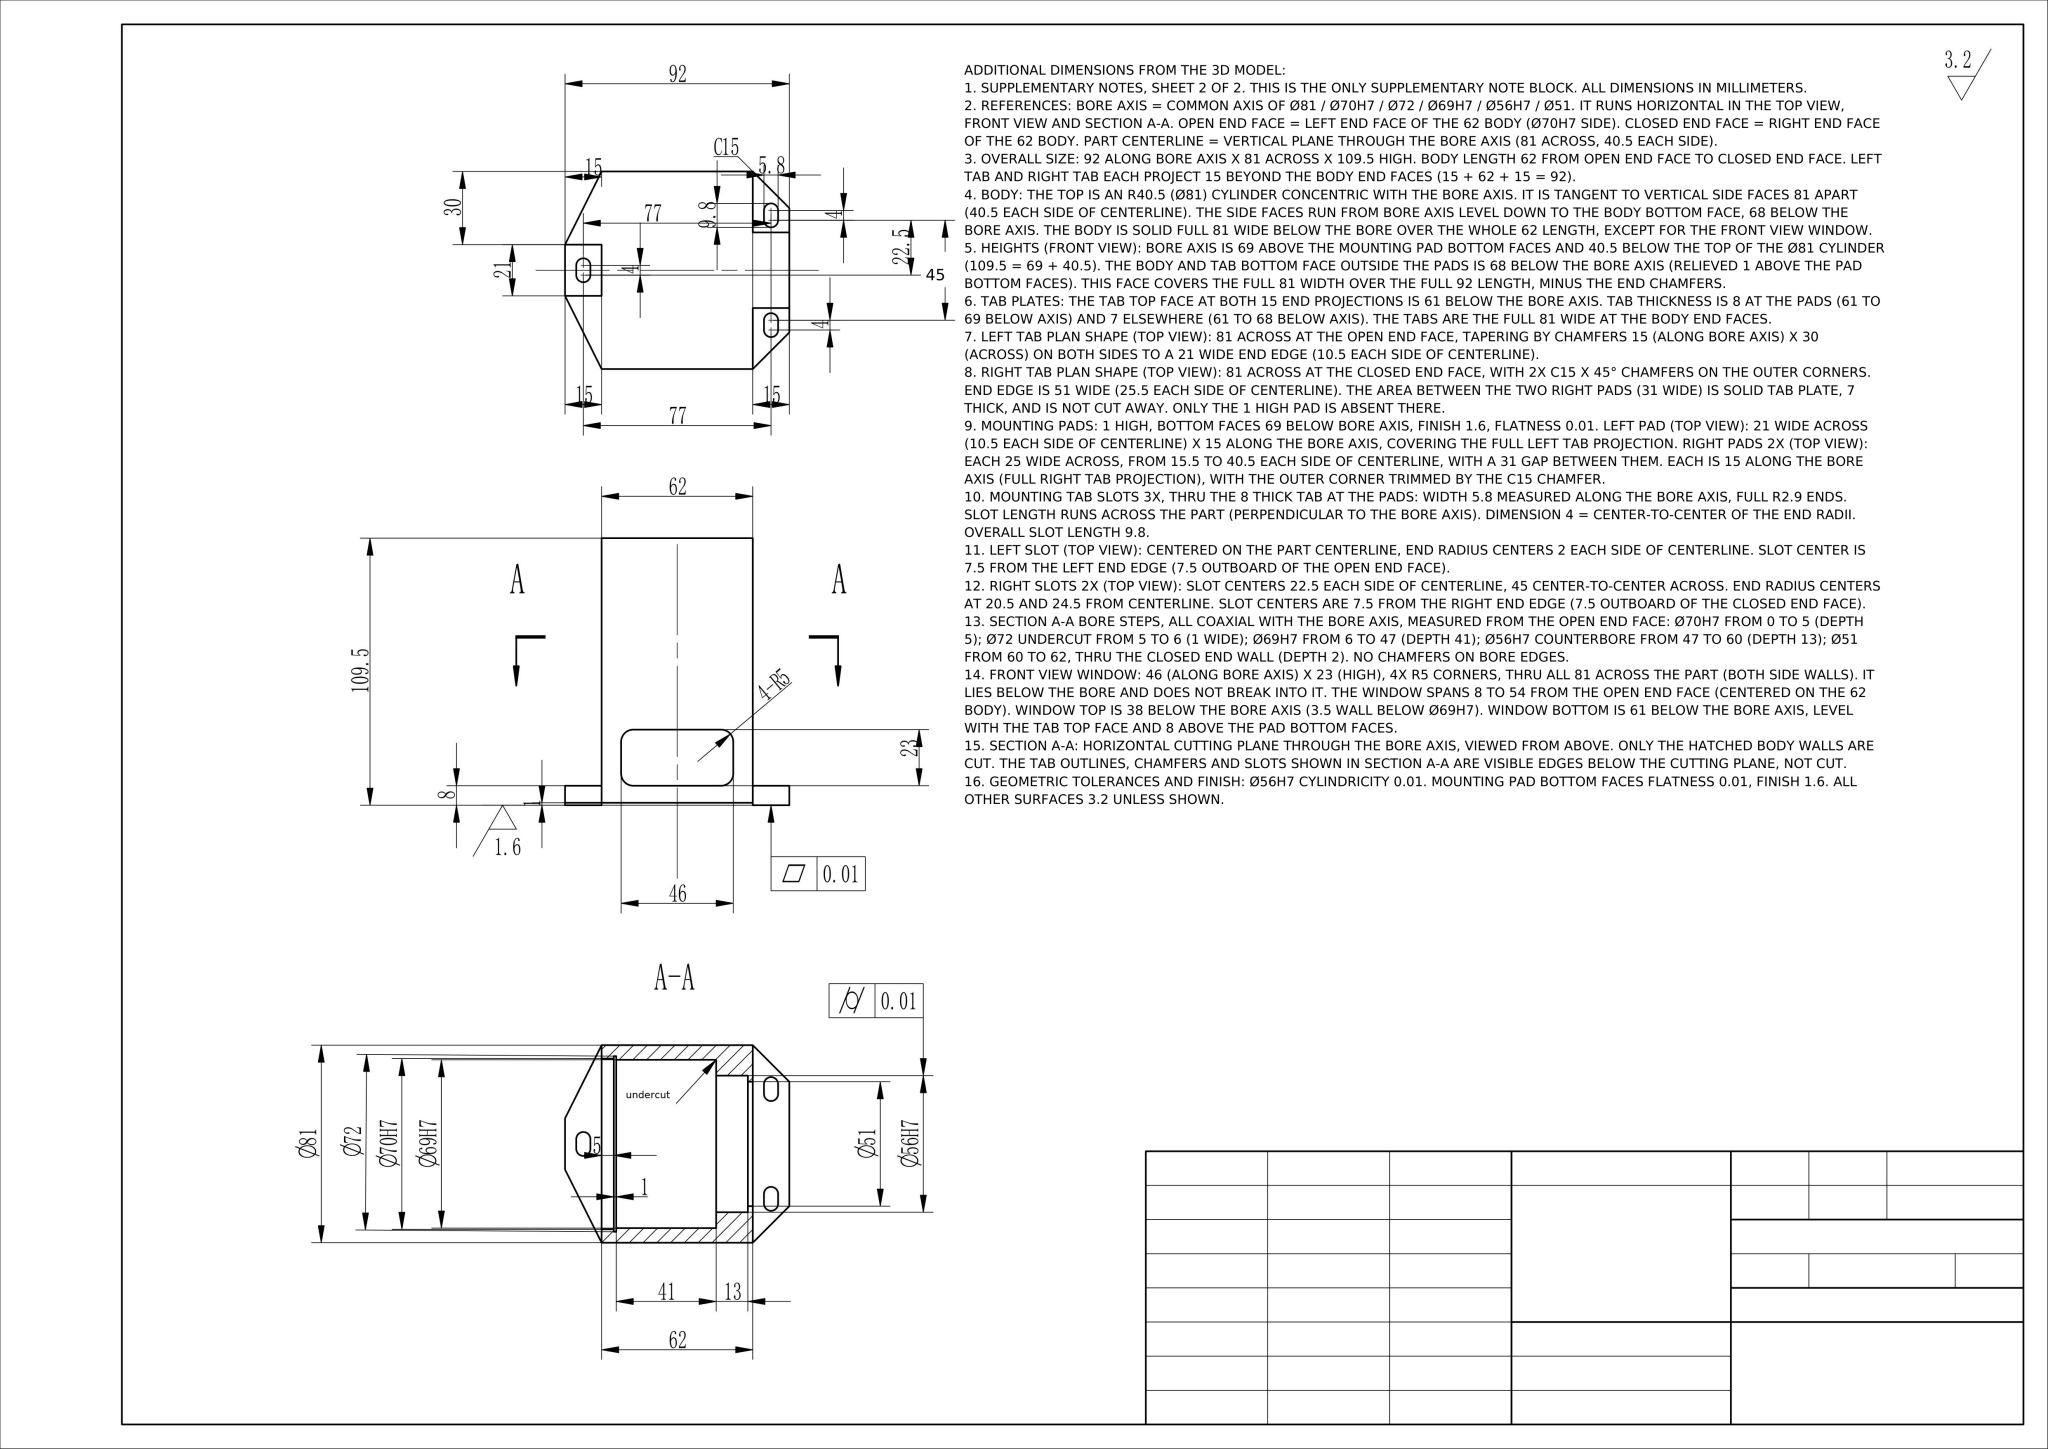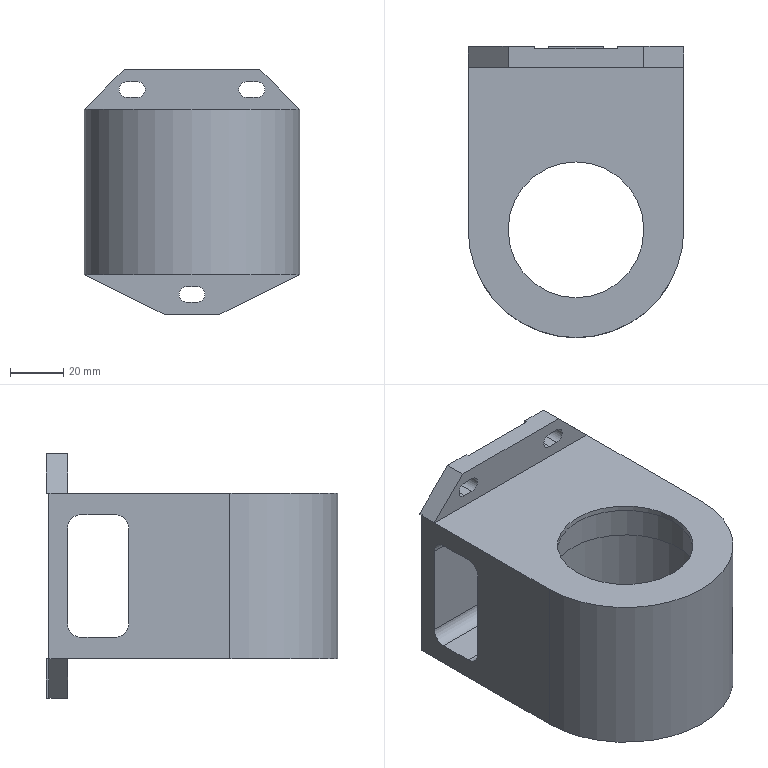Part | NX | mm | 1 solid | 53 faces | box 81 x 109.5 x 92 mm | volume 216484 mm3 | plane 37 | cylinder 16 | commonest cylinder face diameters 5.8 x6 10 x4 69 x1 72 x1 70 x1 81 x1 51 x1 56 x1